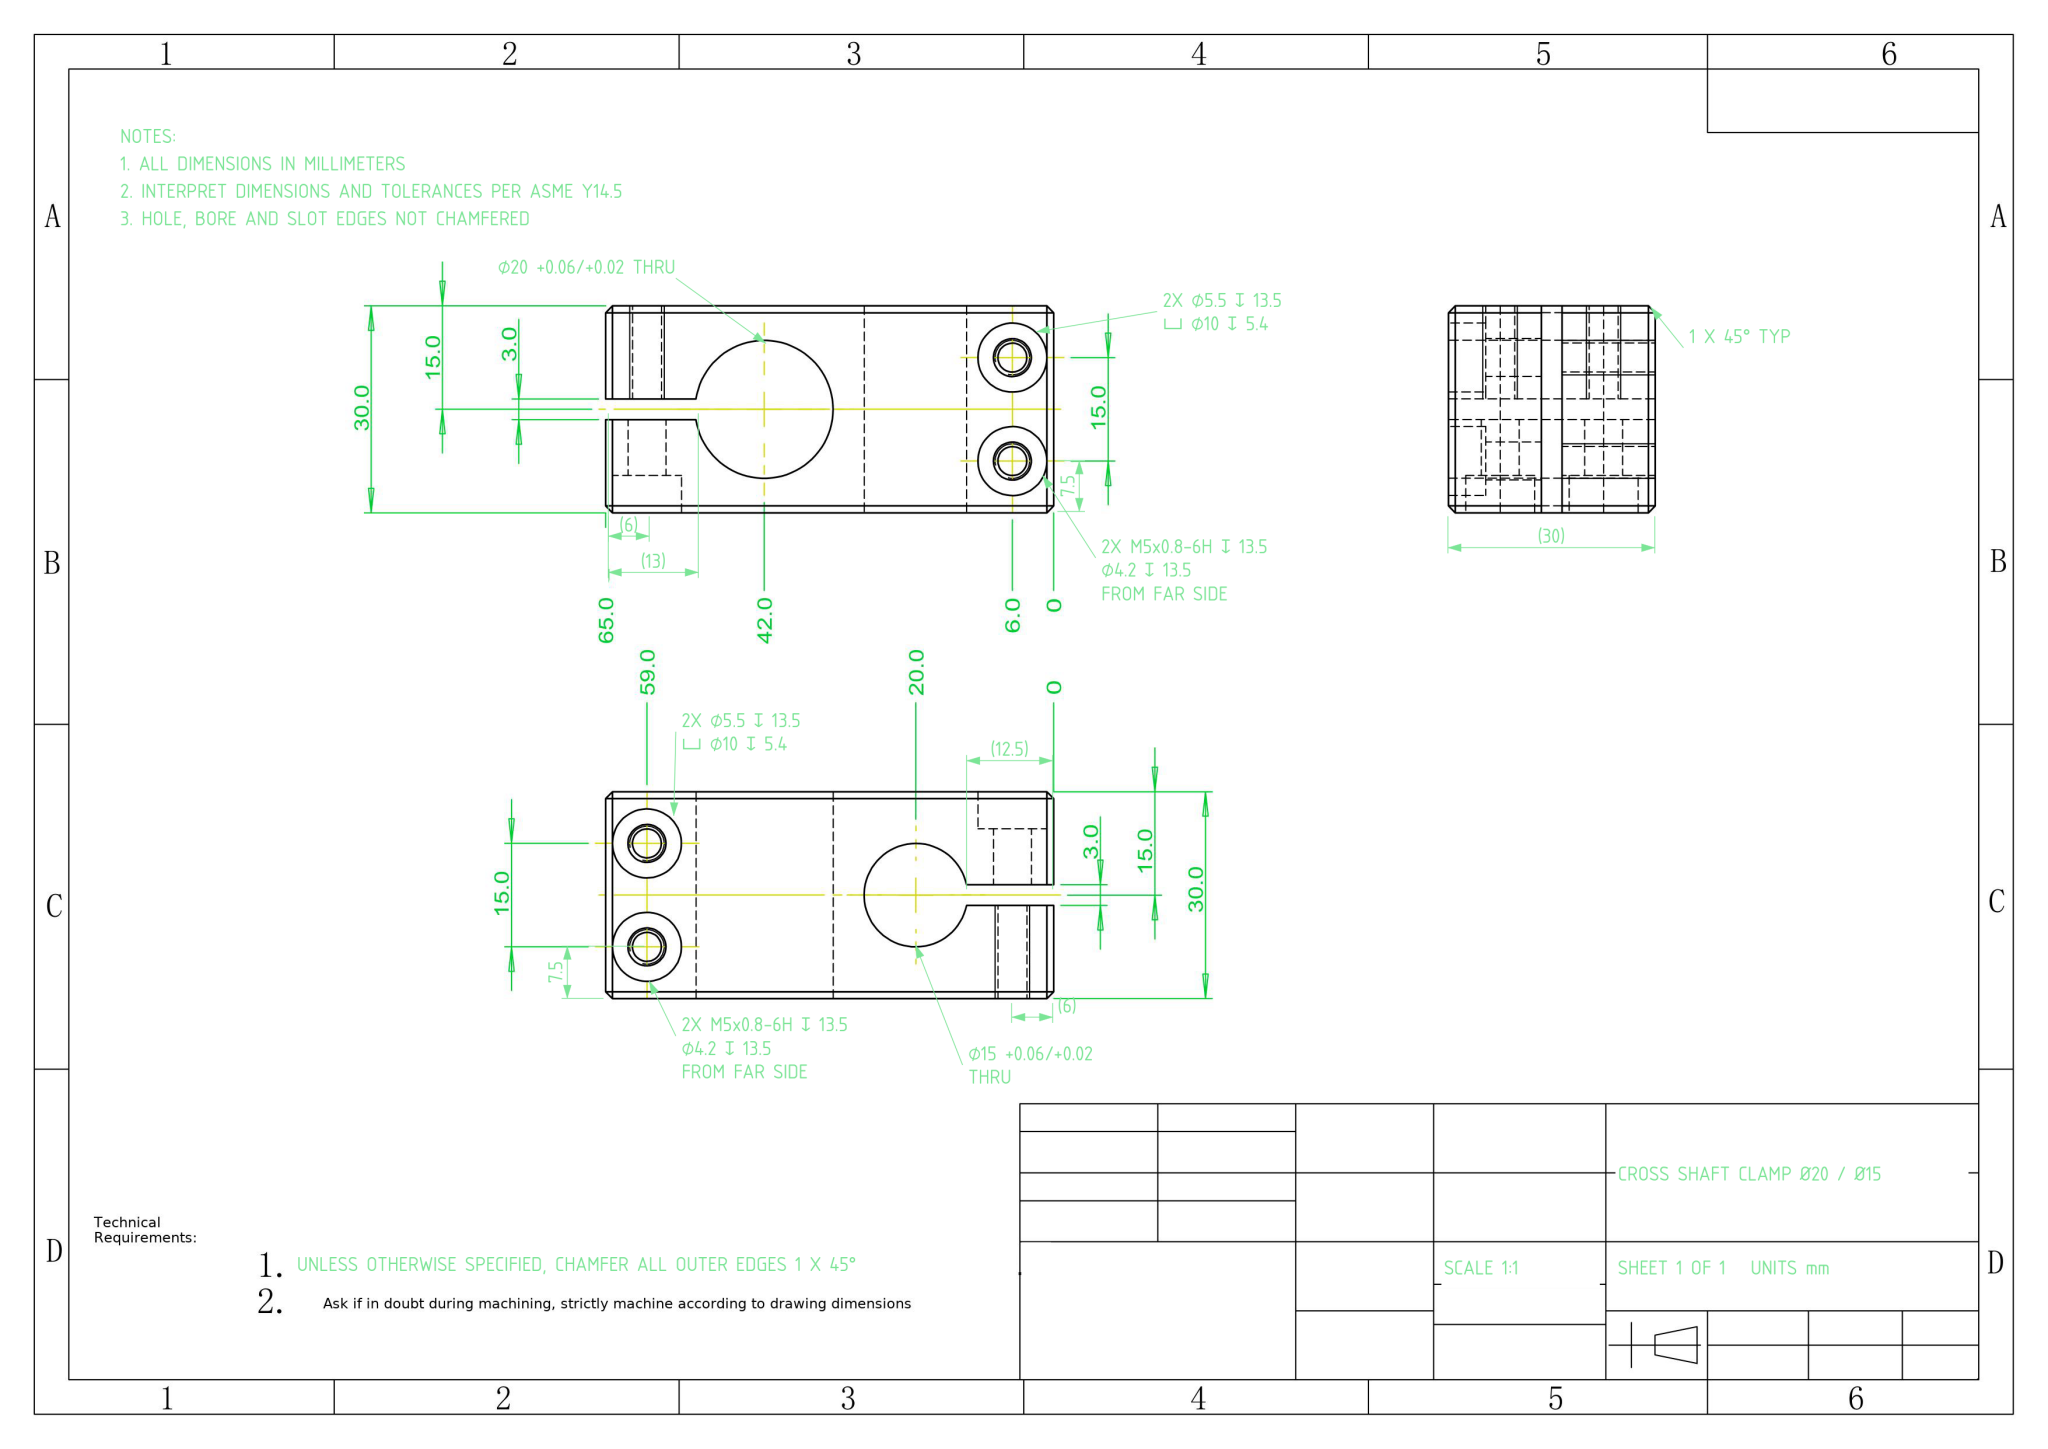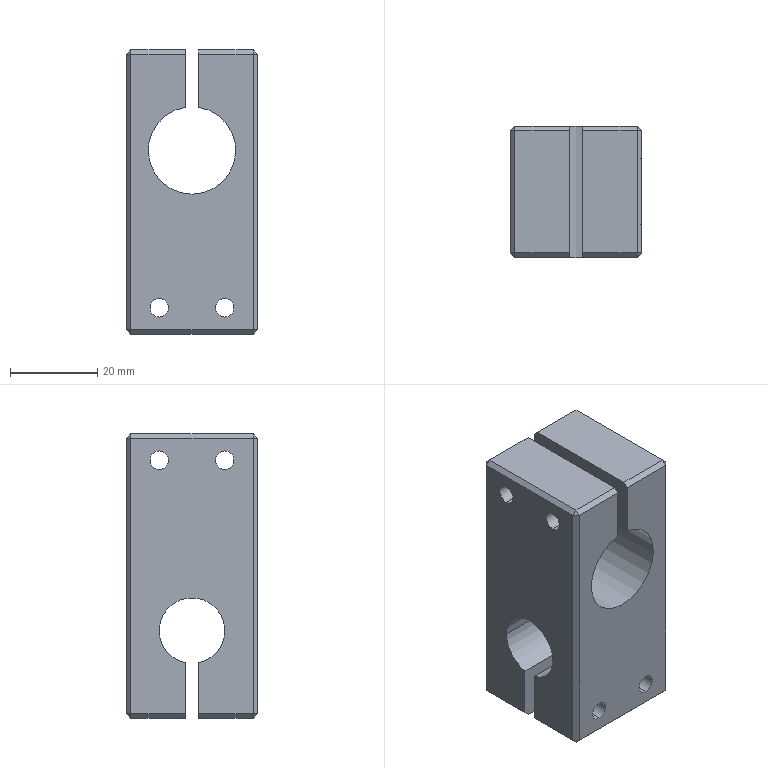Part | NX | mm | 1 solid | 68 faces | box 30 x 30 x 65 mm | volume 38018 mm3 | plane 40 | cylinder 28 | commonest cylinder face diameters 4.2 x8 10 x8 5.5 x8 15 x3 20 x1